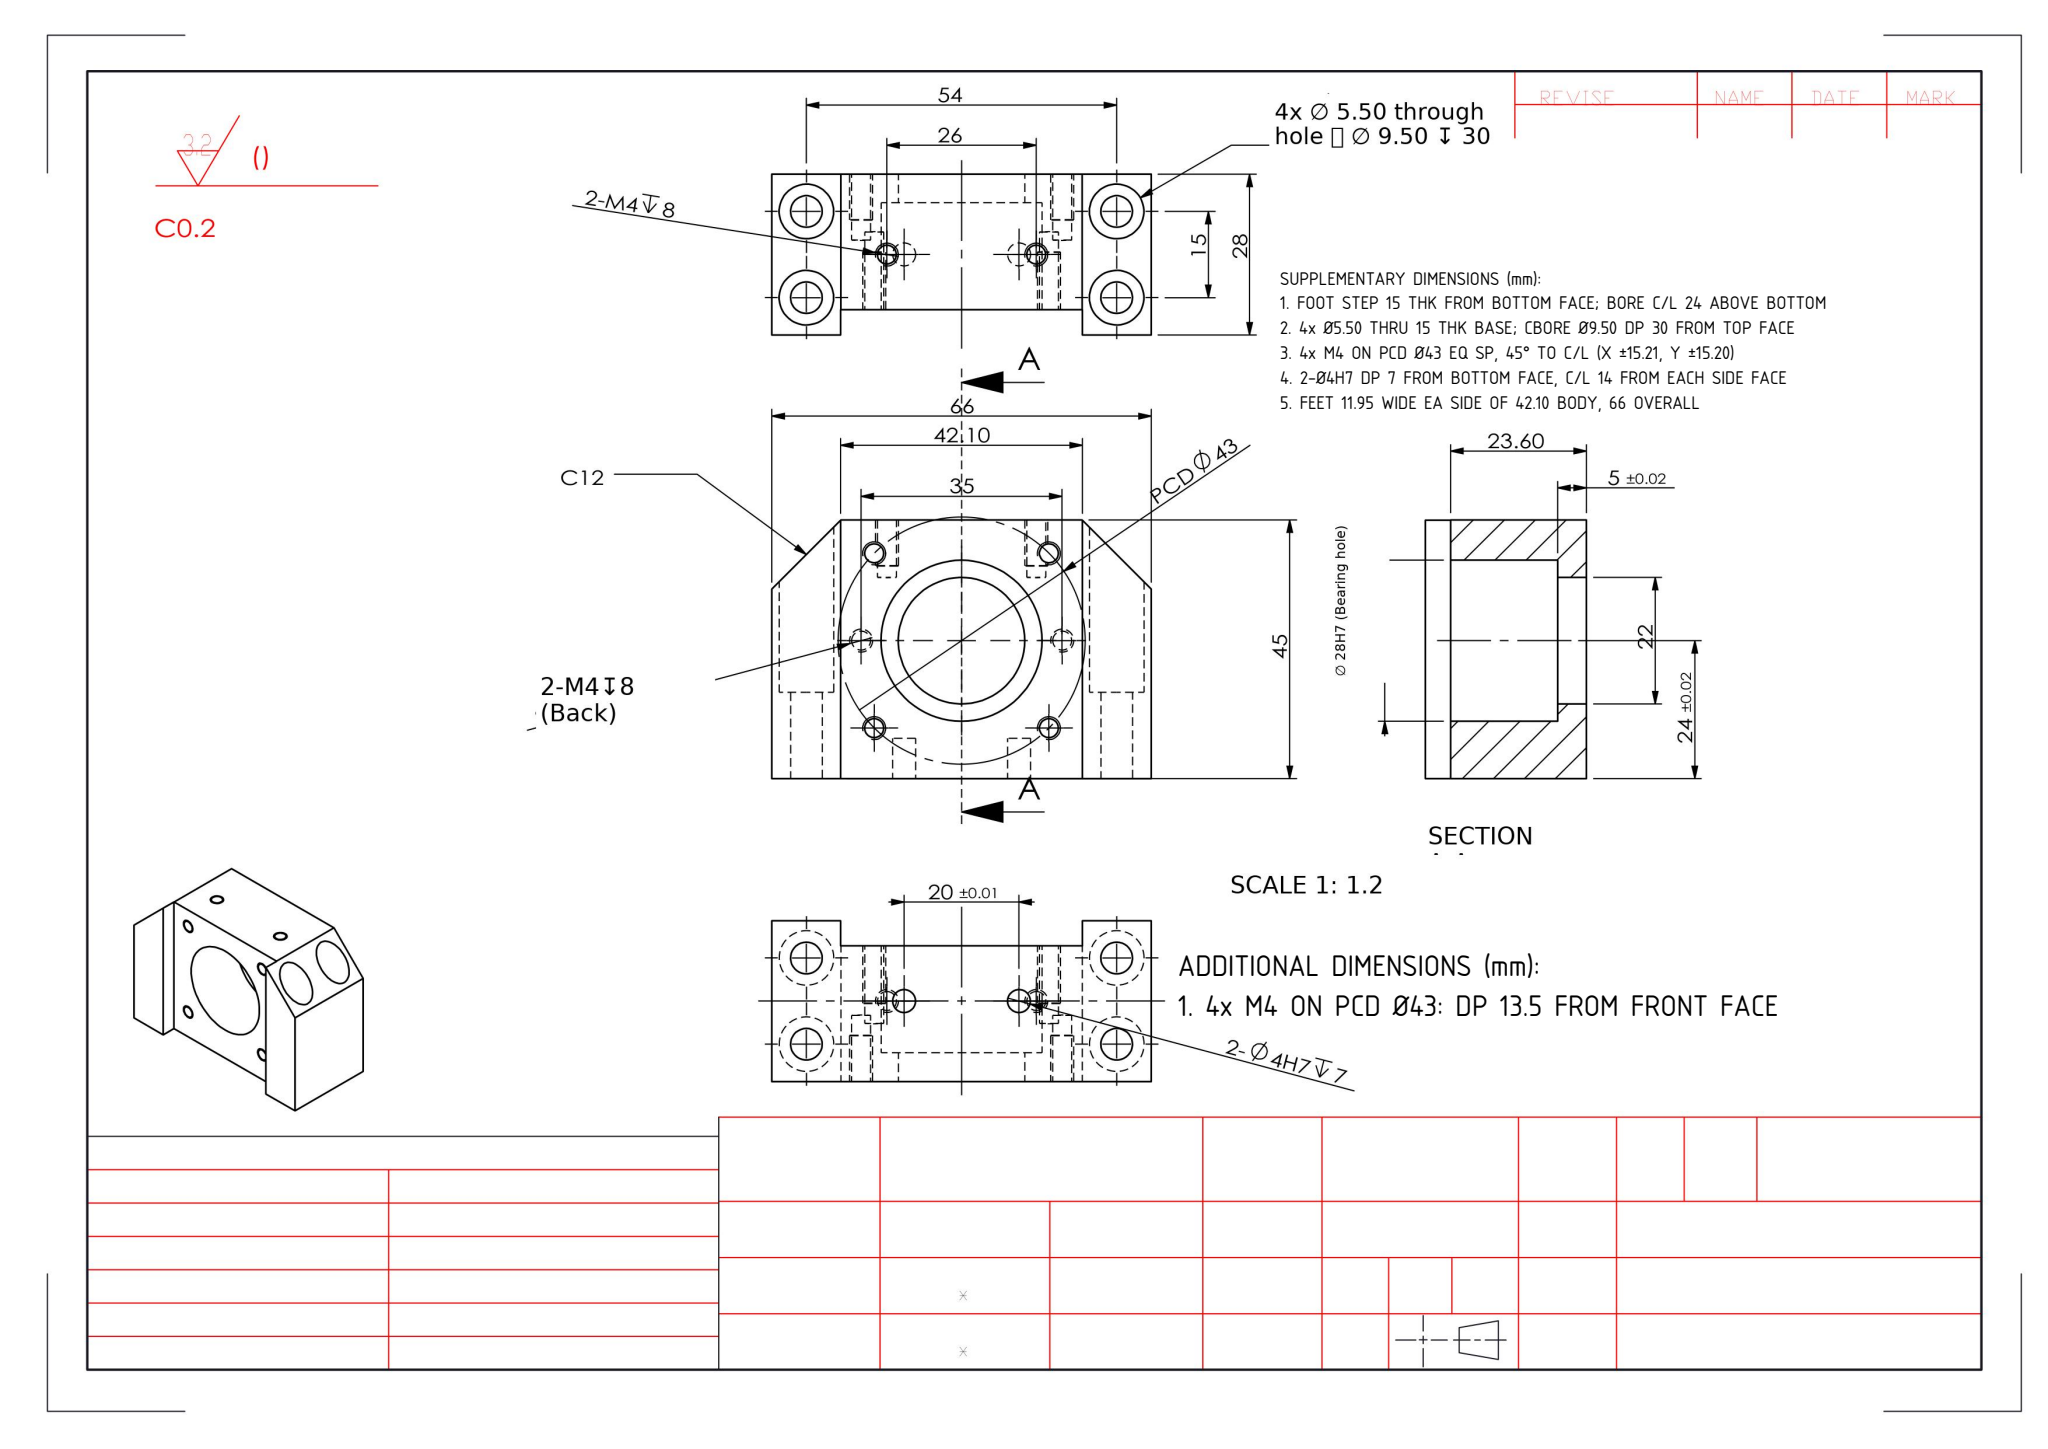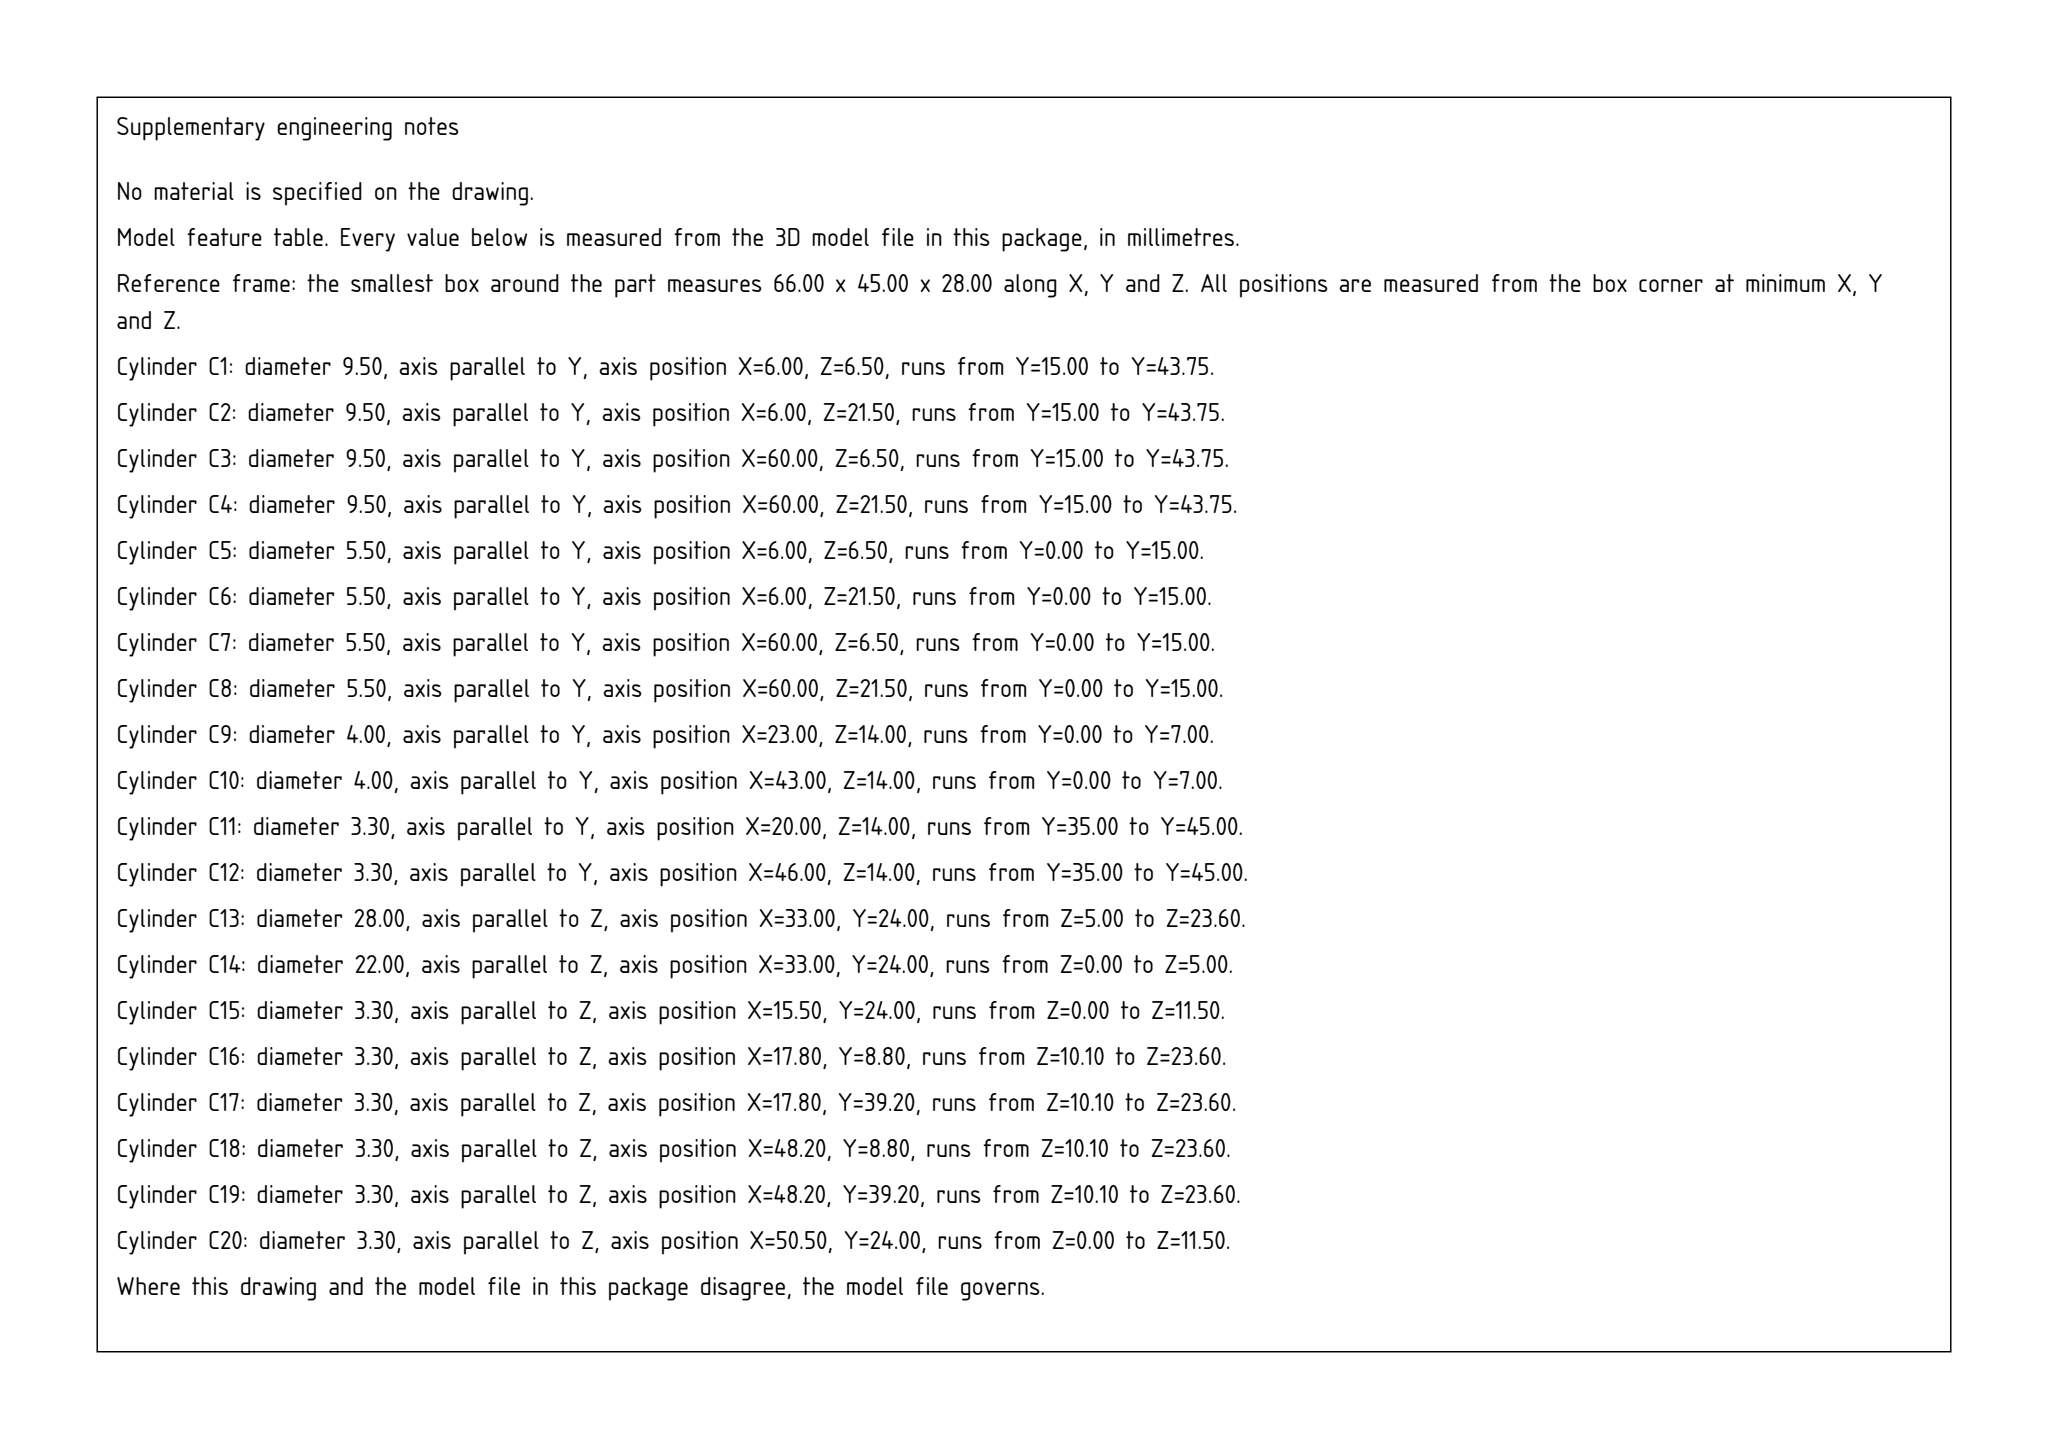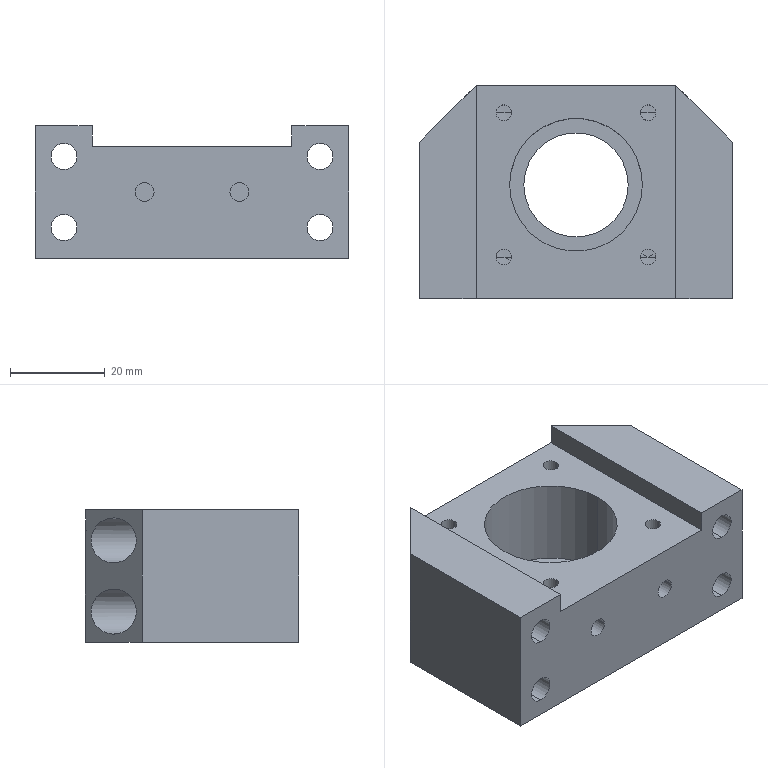Part | SolidWorks | mm | 1 solid | 75 faces | box 66 x 45 x 28 mm | volume 48212 mm3 | cylinder 40 | plane 19 | cone 16 | commonest cylinder face diameters 3.3 x16 9.5 x8 5.5 x8 4 x4 22 x2 28 x2
build123d program:
from build123d import *

# Parameters (mm, degrees)
SKETCH1_W                                       = 66
SKETCH1_H                                       = 45
EXTRUDE1_DEPTH                                  = 28
CHAMFER1_SIZE                                   = 12
M5_HEX_SOCKET_HEAD_CAP_SCREW_CBORE1_D           = 5.5
M5_HEX_SOCKET_HEAD_CAP_SCREW_CBORE1_CBORE_D     = 9.5
M5_HEX_SOCKET_HEAD_CAP_SCREW_CBORE1_CBORE_DEPTH = 30
SKETCH8_W                                       = 42.1
SKETCH8_H                                       = 52.723
EXTRUDE2_DEPTH                                  = 4.4
M4_TAPPED_HOLE1_D                               = 3.3
M4_TAPPED_HOLE1_DEPTH                           = 13.5
M4_TAPPED_HOLE1_TIP                             = 0.07204
SKETCH9_R                                       = 2
EXTRUDE3_DEPTH                                  = 7
M4_TAPPED_HOLE2_D                               = 3.3
M4_TAPPED_HOLE2_DEPTH                           = 10
M4_TAPPED_HOLE2_TIP                             = 0.07204
M4_TAPPED_HOLE3_D                               = 3.3
M4_TAPPED_HOLE3_DEPTH                           = 11.5
M4_TAPPED_HOLE3_TIP                             = 0.07204


with BuildPart() as part:
    # Sketch1 → Extrude1 (new body)
    with BuildSketch(Plane.XY):
        with Locations((0, 22.5)):
            Rectangle(SKETCH1_W, SKETCH1_H)
    extrude(amount=EXTRUDE1_DEPTH)

    # Chamfer1
    chamfer1_edges = [part.edges().sort_by_distance(p)[0] for p in [
        (-33, 45, 14),
        (33, 45, 14),
    ]]
    chamfer(chamfer1_edges, length=CHAMFER1_SIZE)

    # Sketch3 → Cut-Revolve1 (revolve, cut)
    with BuildSketch(Plane(origin=(0, 0, 0), x_dir=(0, 0, -1), z_dir=(1, 0, 0)), mode=Mode.PRIVATE) as cut_revolve1_sk:
        Polygon((0, 35), (-5, 35), (-5, 38), (-31.16, 38), (-31.16, 24), (0, 24), align=None)
    revolve(cut_revolve1_sk.sketch.rotate(Axis((0, 24, 49.469), (0, 0, -1)), 90), axis=Axis((0, 24, 49.469), (0, 0, -1)), mode=Mode.SUBTRACT)

    # M5 Hex Socket Head Cap Screw CBORE1 (through all)
    with Locations(Plane(origin=(-27, 45, 6.5), x_dir=(0, 0, 1), z_dir=(0, 1, 0))):
        with Locations((0, 0), (15, 0), (0, 54), (15, 54)):
            CounterBoreHole(M5_HEX_SOCKET_HEAD_CAP_SCREW_CBORE1_D / 2, M5_HEX_SOCKET_HEAD_CAP_SCREW_CBORE1_CBORE_D / 2, M5_HEX_SOCKET_HEAD_CAP_SCREW_CBORE1_CBORE_DEPTH)

    # Sketch8 → Extrude2 (cut)
    with BuildSketch(Plane.XY.offset(28)):
        with Locations((0, 24)):
            Rectangle(SKETCH8_W, SKETCH8_H)
    extrude(amount=-EXTRUDE2_DEPTH, mode=Mode.SUBTRACT)

    # M4 Tapped Hole1
    with Locations(Plane(origin=(-15.203, 39.203, 23.6), x_dir=(1, 0, 0), z_dir=(0, 0, 1))):
        with Locations((0, 0), (30.406, 0), (30.406, -30.406), (0, -30.406)):
            Hole(M4_TAPPED_HOLE1_D / 2, depth=M4_TAPPED_HOLE1_DEPTH)
            with Locations((0, 0, -(M4_TAPPED_HOLE1_DEPTH + M4_TAPPED_HOLE1_TIP / 2))):  # 175° drill point
                Cone(0, M4_TAPPED_HOLE1_D / 2, M4_TAPPED_HOLE1_TIP, mode=Mode.SUBTRACT)

    # Sketch9 → Extrude3 (cut)
    with BuildSketch(Plane.XZ):
        with Locations((-10, 14)):
            Circle(SKETCH9_R)
        with Locations((10, 14)):
            Circle(SKETCH9_R)
    extrude(amount=-EXTRUDE3_DEPTH, mode=Mode.SUBTRACT)

    # M4 Tapped Hole2
    with Locations(Plane(origin=(-13, 45, 14), x_dir=(0, 0, 1), z_dir=(0, 1, 0))):
        with Locations((0, 0), (0, 26)):
            Hole(M4_TAPPED_HOLE2_D / 2, depth=M4_TAPPED_HOLE2_DEPTH)
            with Locations((0, 0, -(M4_TAPPED_HOLE2_DEPTH + M4_TAPPED_HOLE2_TIP / 2))):  # 175° drill point
                Cone(0, M4_TAPPED_HOLE2_D / 2, M4_TAPPED_HOLE2_TIP, mode=Mode.SUBTRACT)

    # M4 Tapped Hole3
    with Locations(Plane(origin=(17.5, 24, 0), x_dir=(-1, 0, 0), z_dir=(0, 0, -1))):
        with Locations((0, 0), (35, 0)):
            Hole(M4_TAPPED_HOLE3_D / 2, depth=M4_TAPPED_HOLE3_DEPTH)
            with Locations((0, 0, -(M4_TAPPED_HOLE3_DEPTH + M4_TAPPED_HOLE3_TIP / 2))):  # 175° drill point
                Cone(0, M4_TAPPED_HOLE3_D / 2, M4_TAPPED_HOLE3_TIP, mode=Mode.SUBTRACT)


solid = part.part